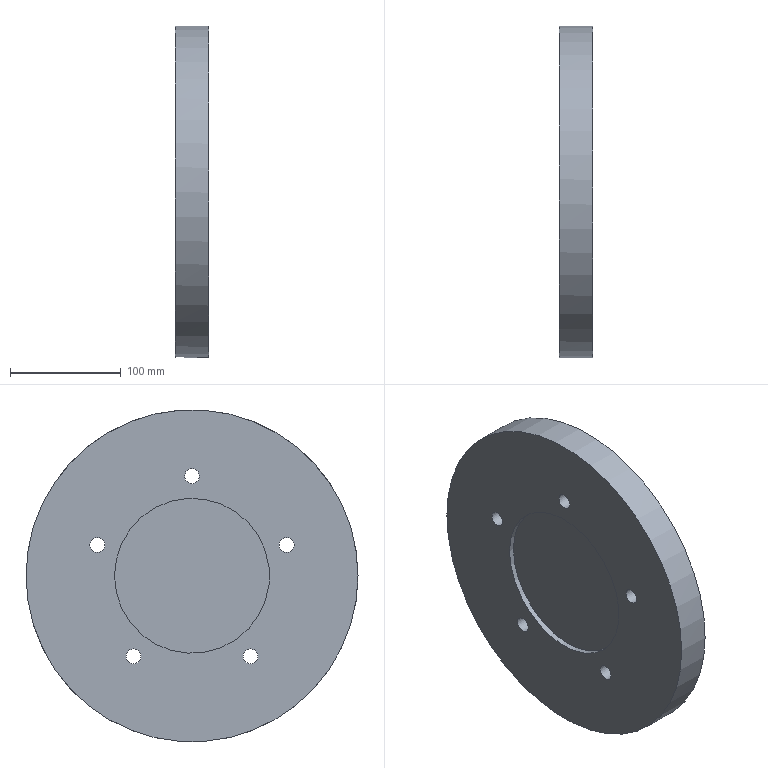Component | NX | FIXTURE_BODY | 1 solid | 40 faces | volume 1978725 mm3 | cylinder 20 | plane 14 | cone 6 | commonest cylinder face diameters 13.5 x5 20 x5 12 x4 6 x4 300 x1 140 x1